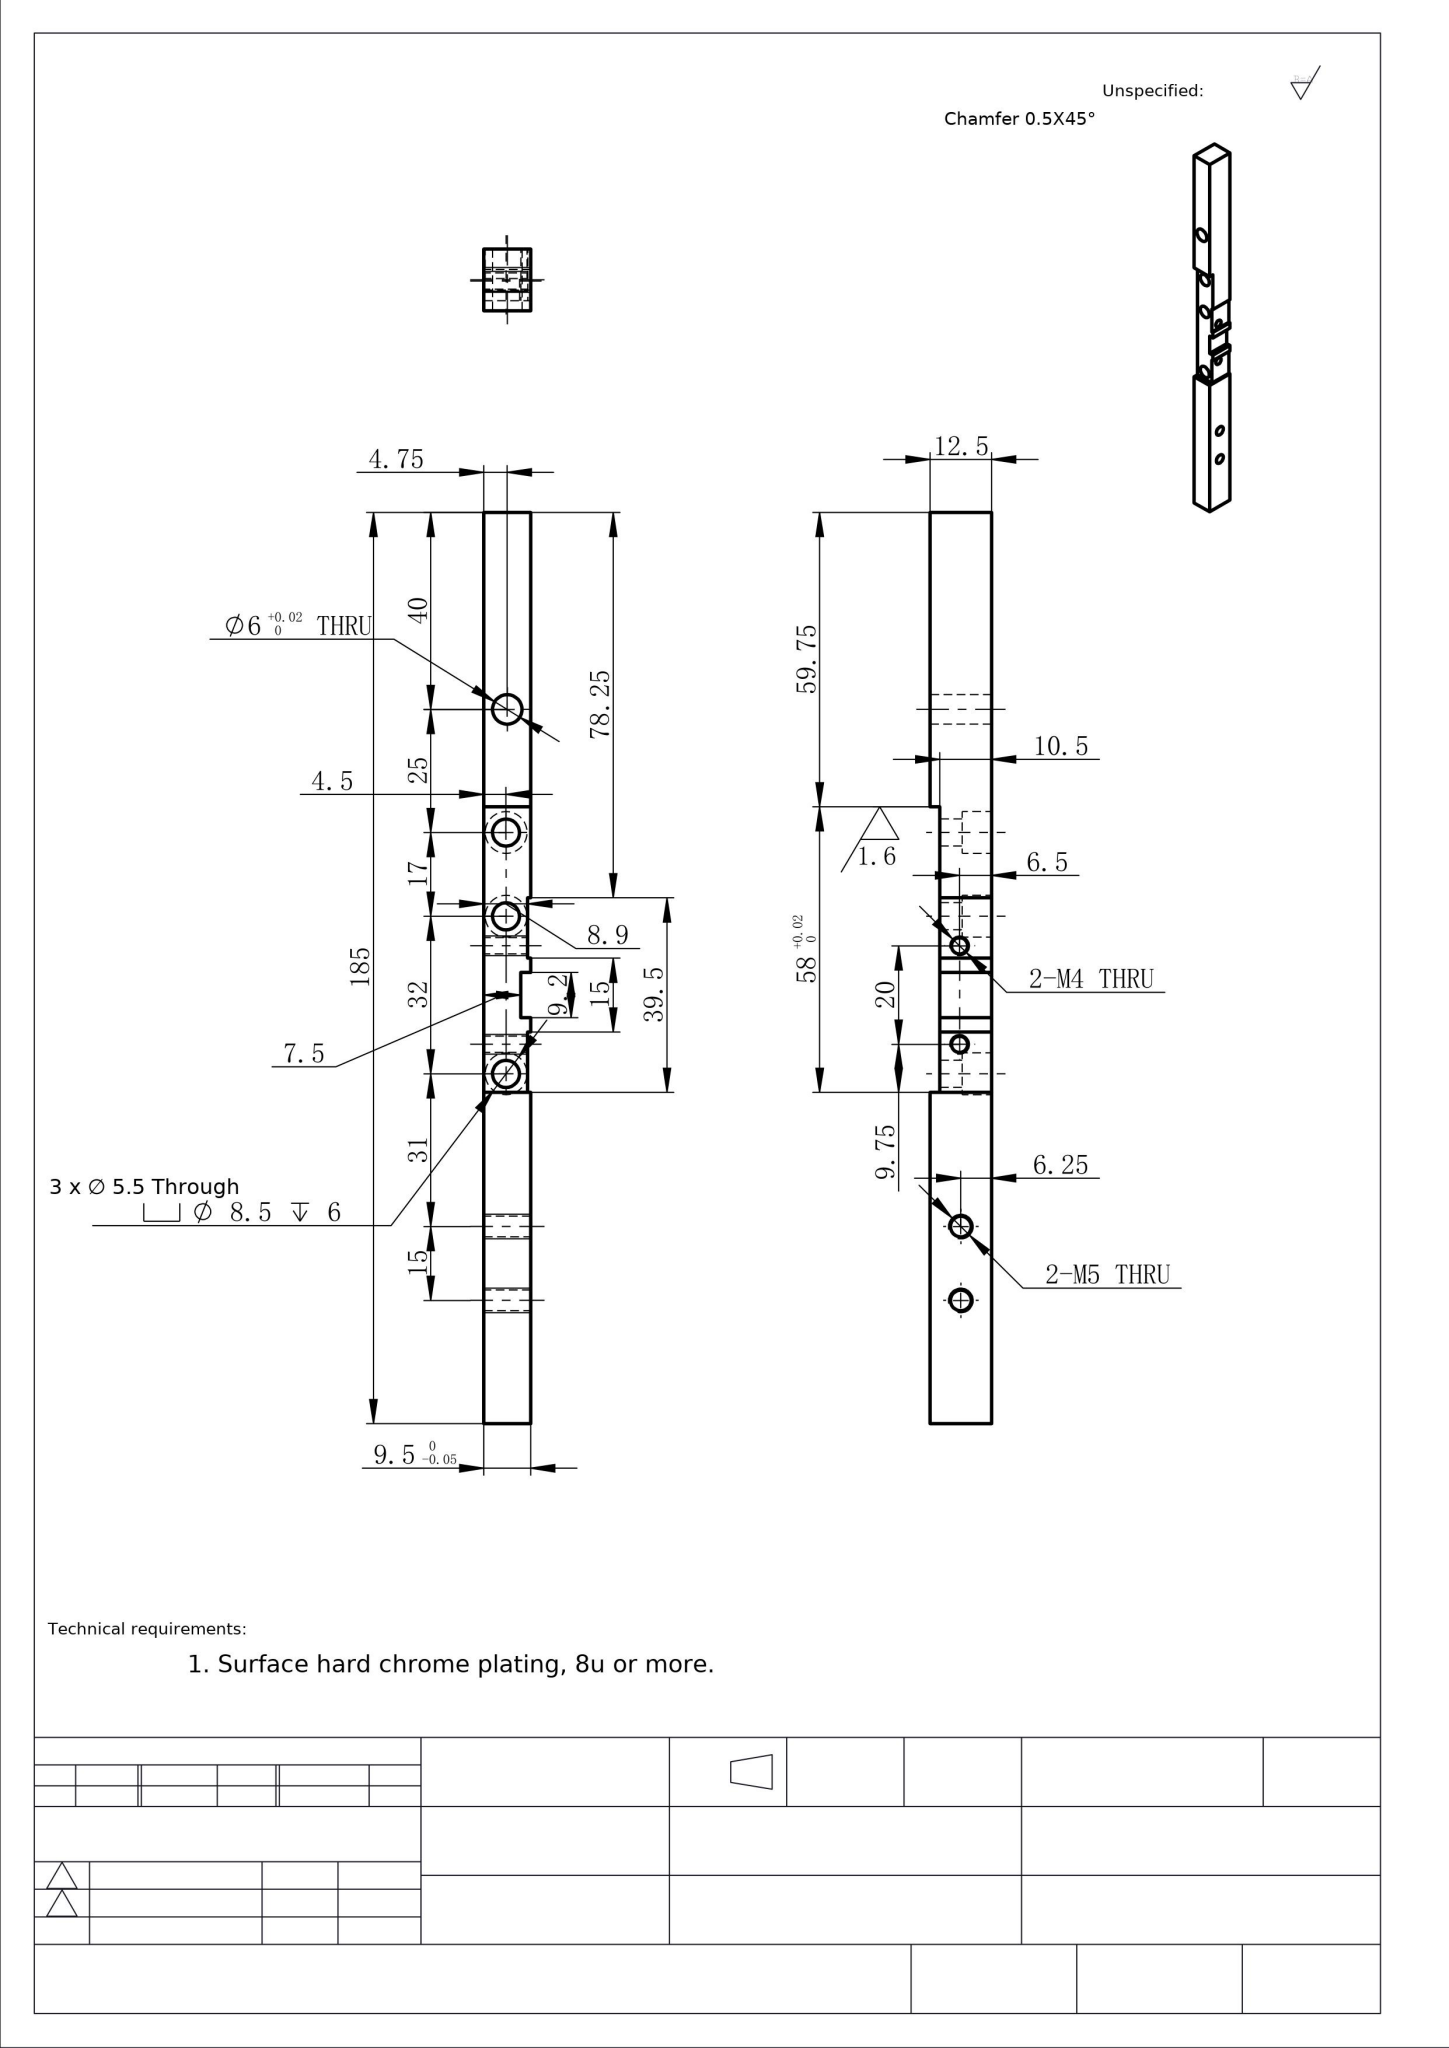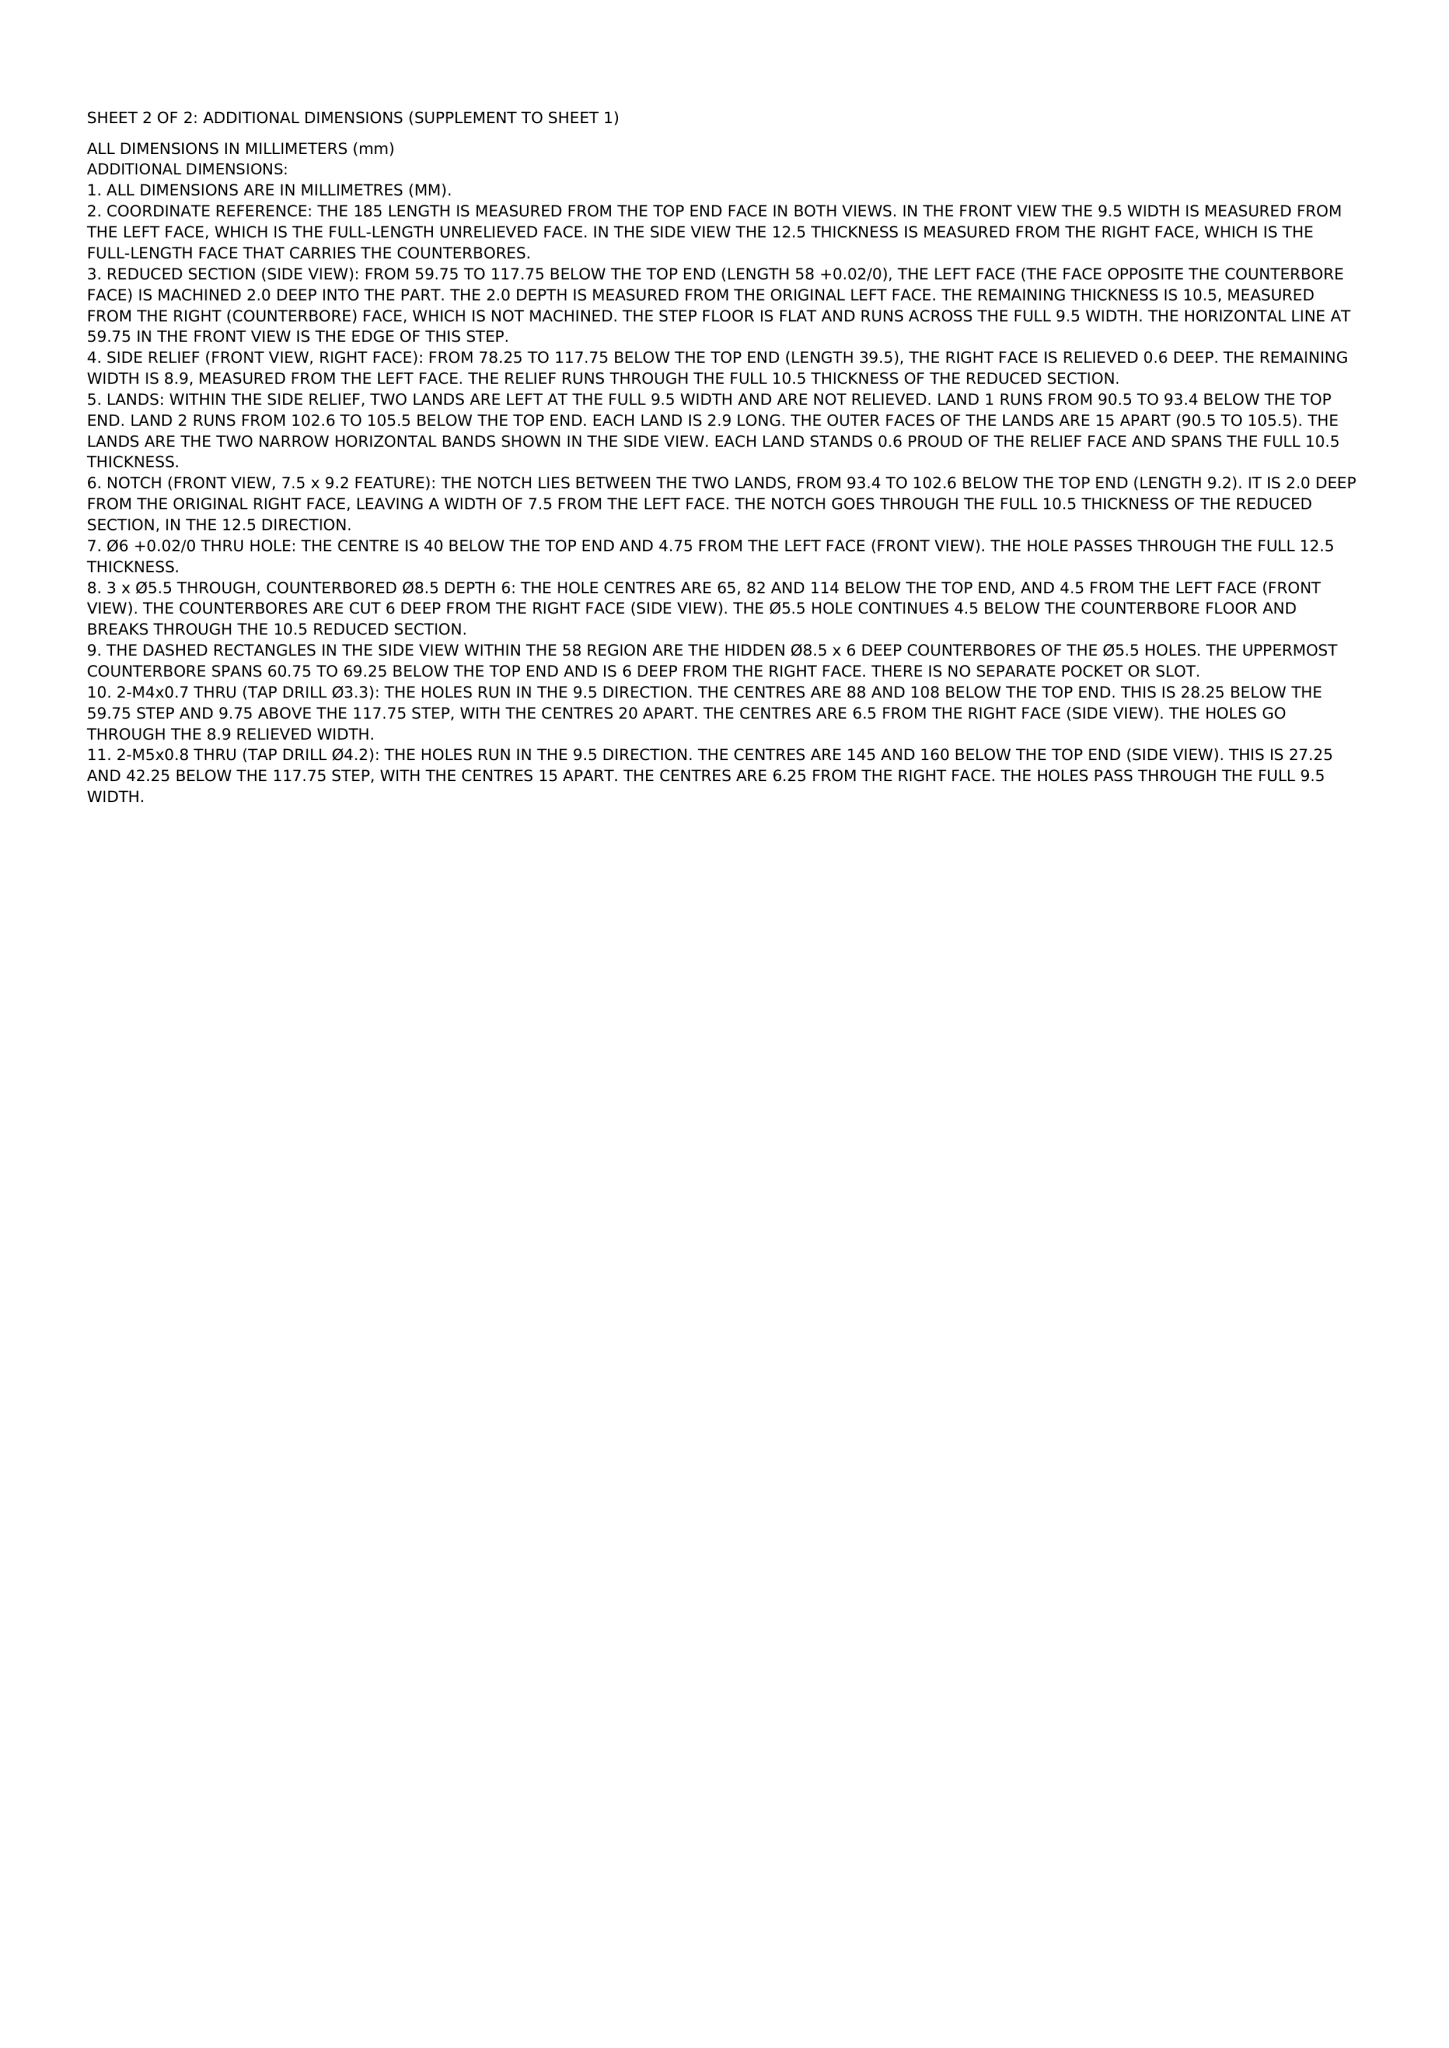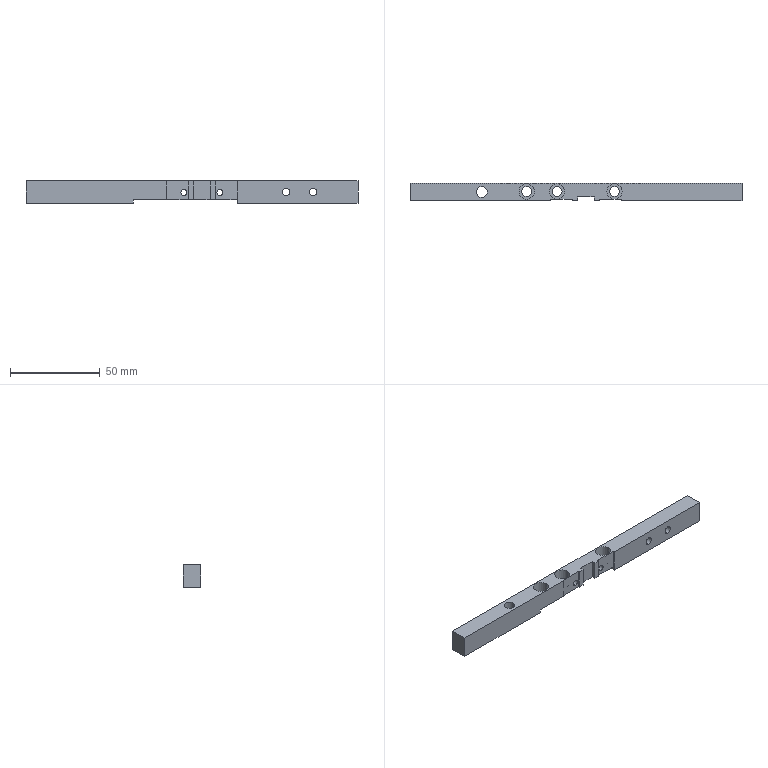Part | NX | mm | 1 solid | 46 faces | box 185 x 9.5 x 12.5 mm | volume 18408 mm3 | plane 24 | cylinder 22 | commonest cylinder face diameters 8.5 x6 5.5 x6 3.3 x4 4.2 x4 6 x2